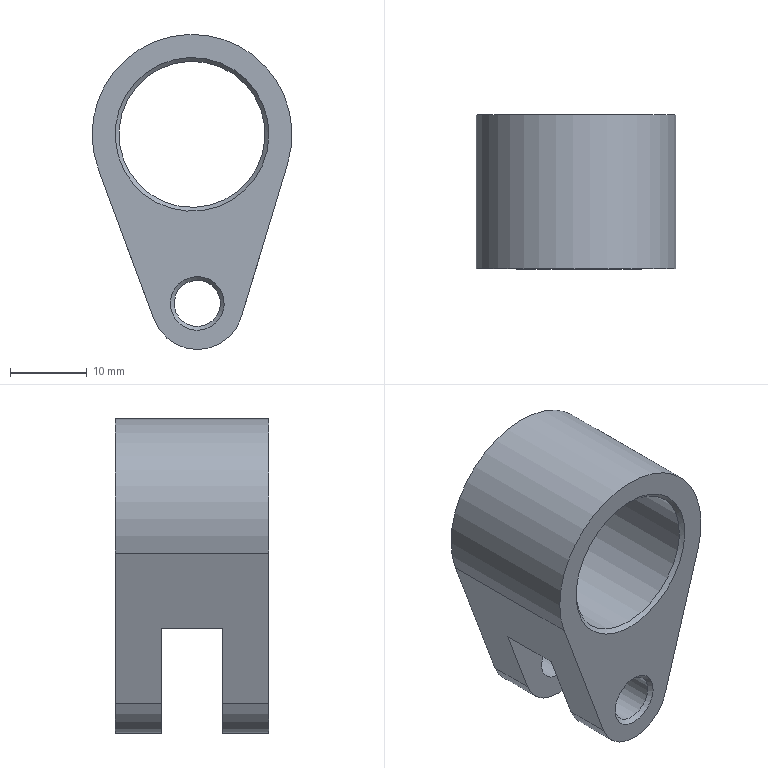Component | NX | 3 | 1 solid | 17 faces | volume 7759 mm3 | plane 7 | cylinder 6 | cone 4 | commonest cylinder face diameters 12 x2 6 x2 26 x1 19 x1